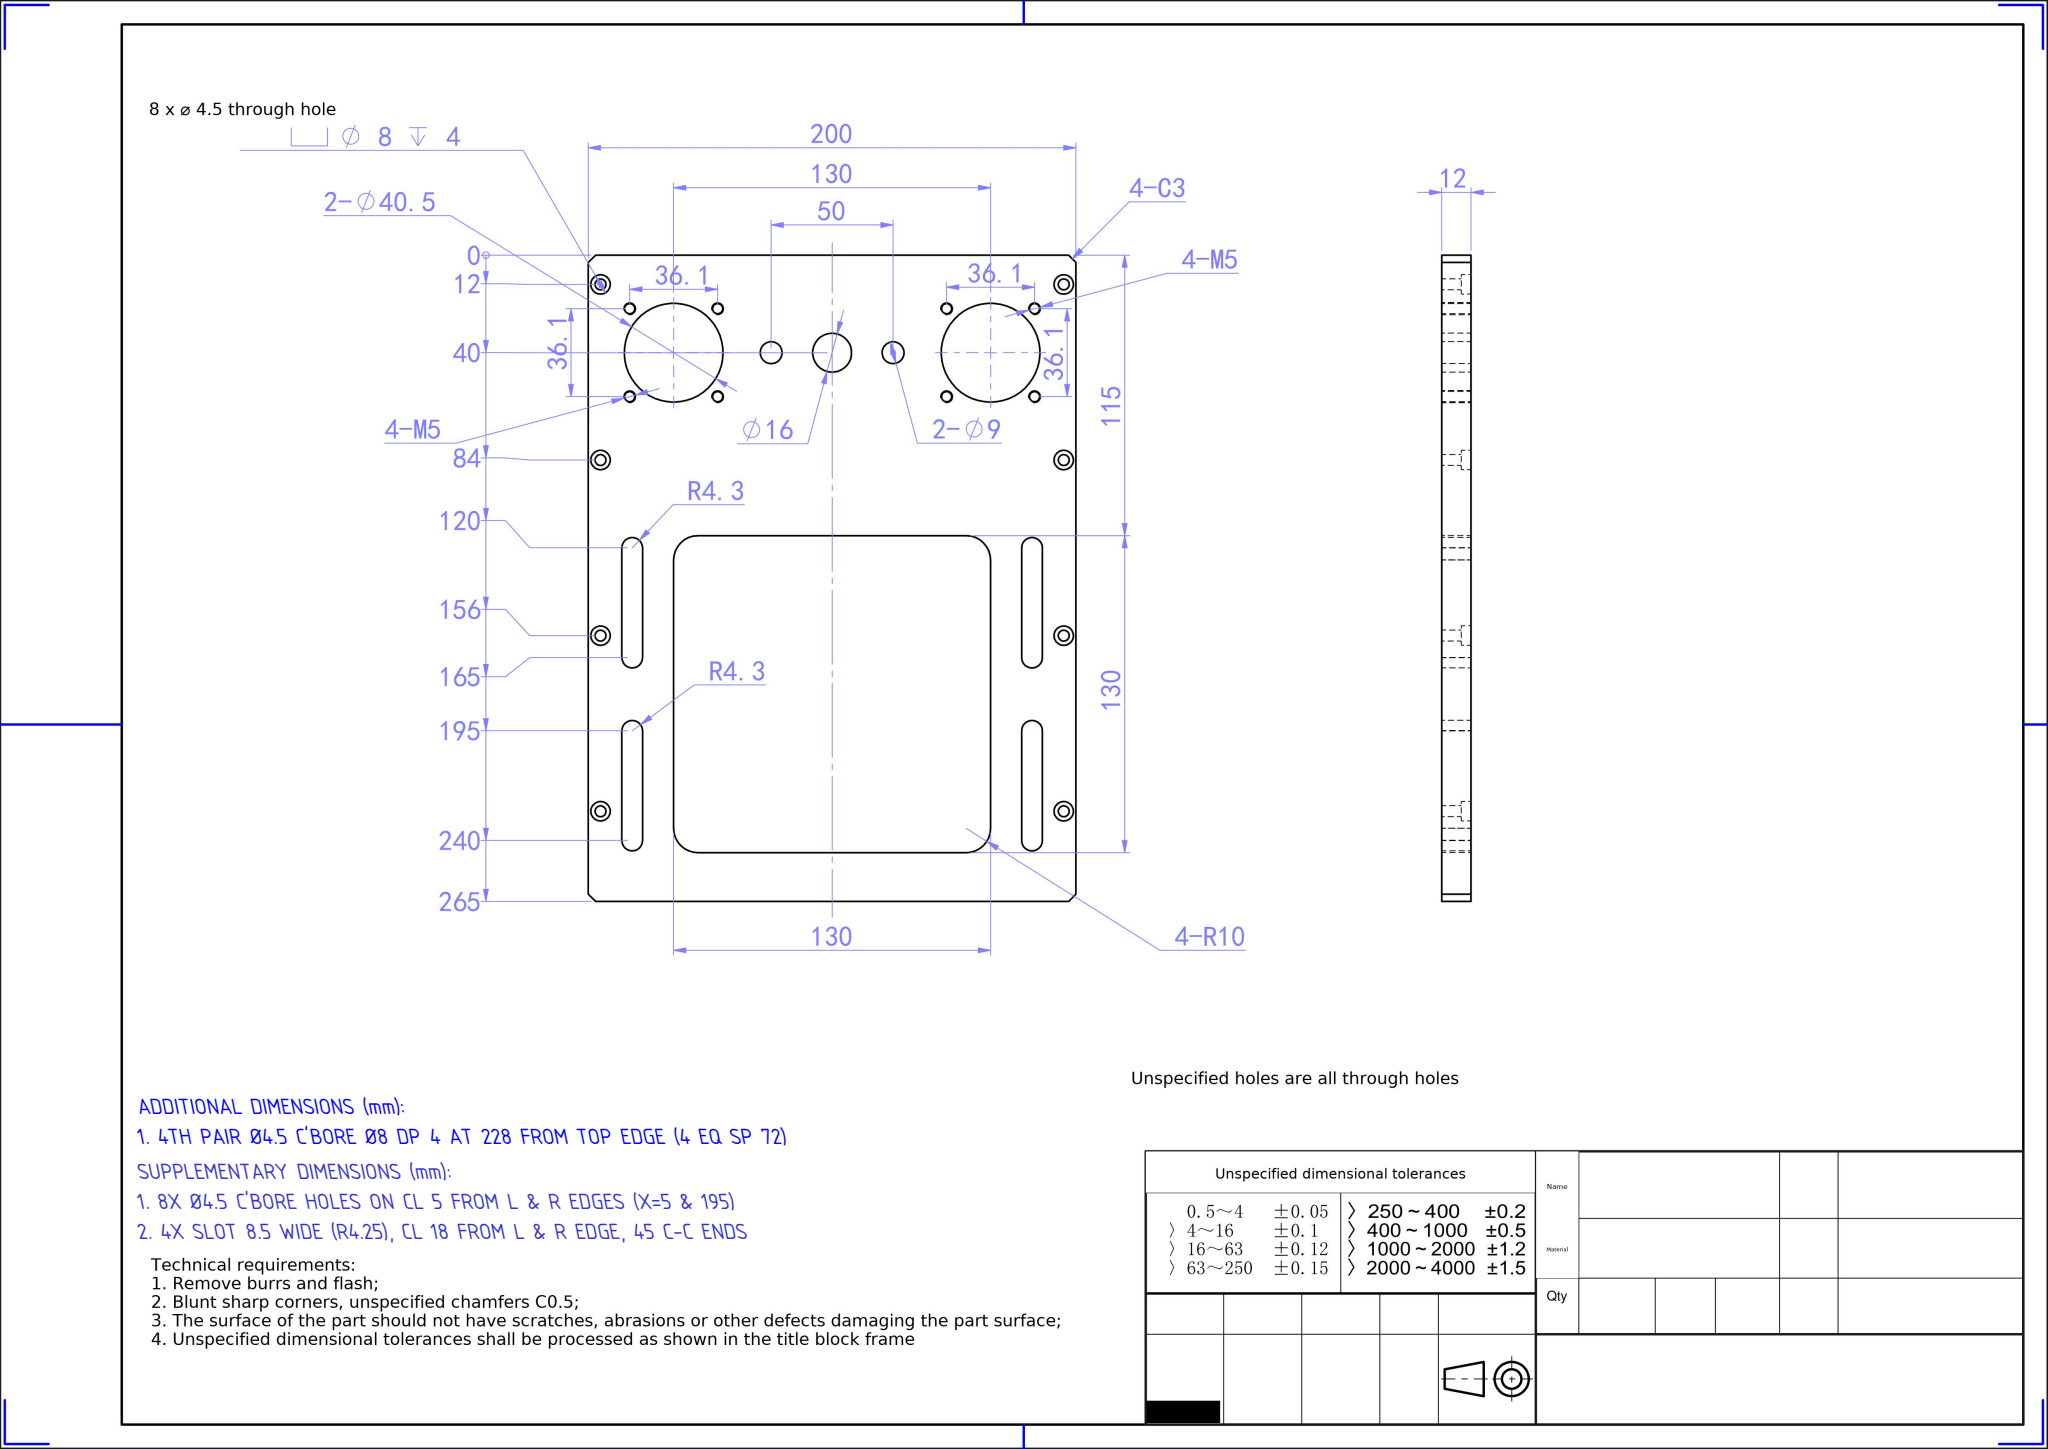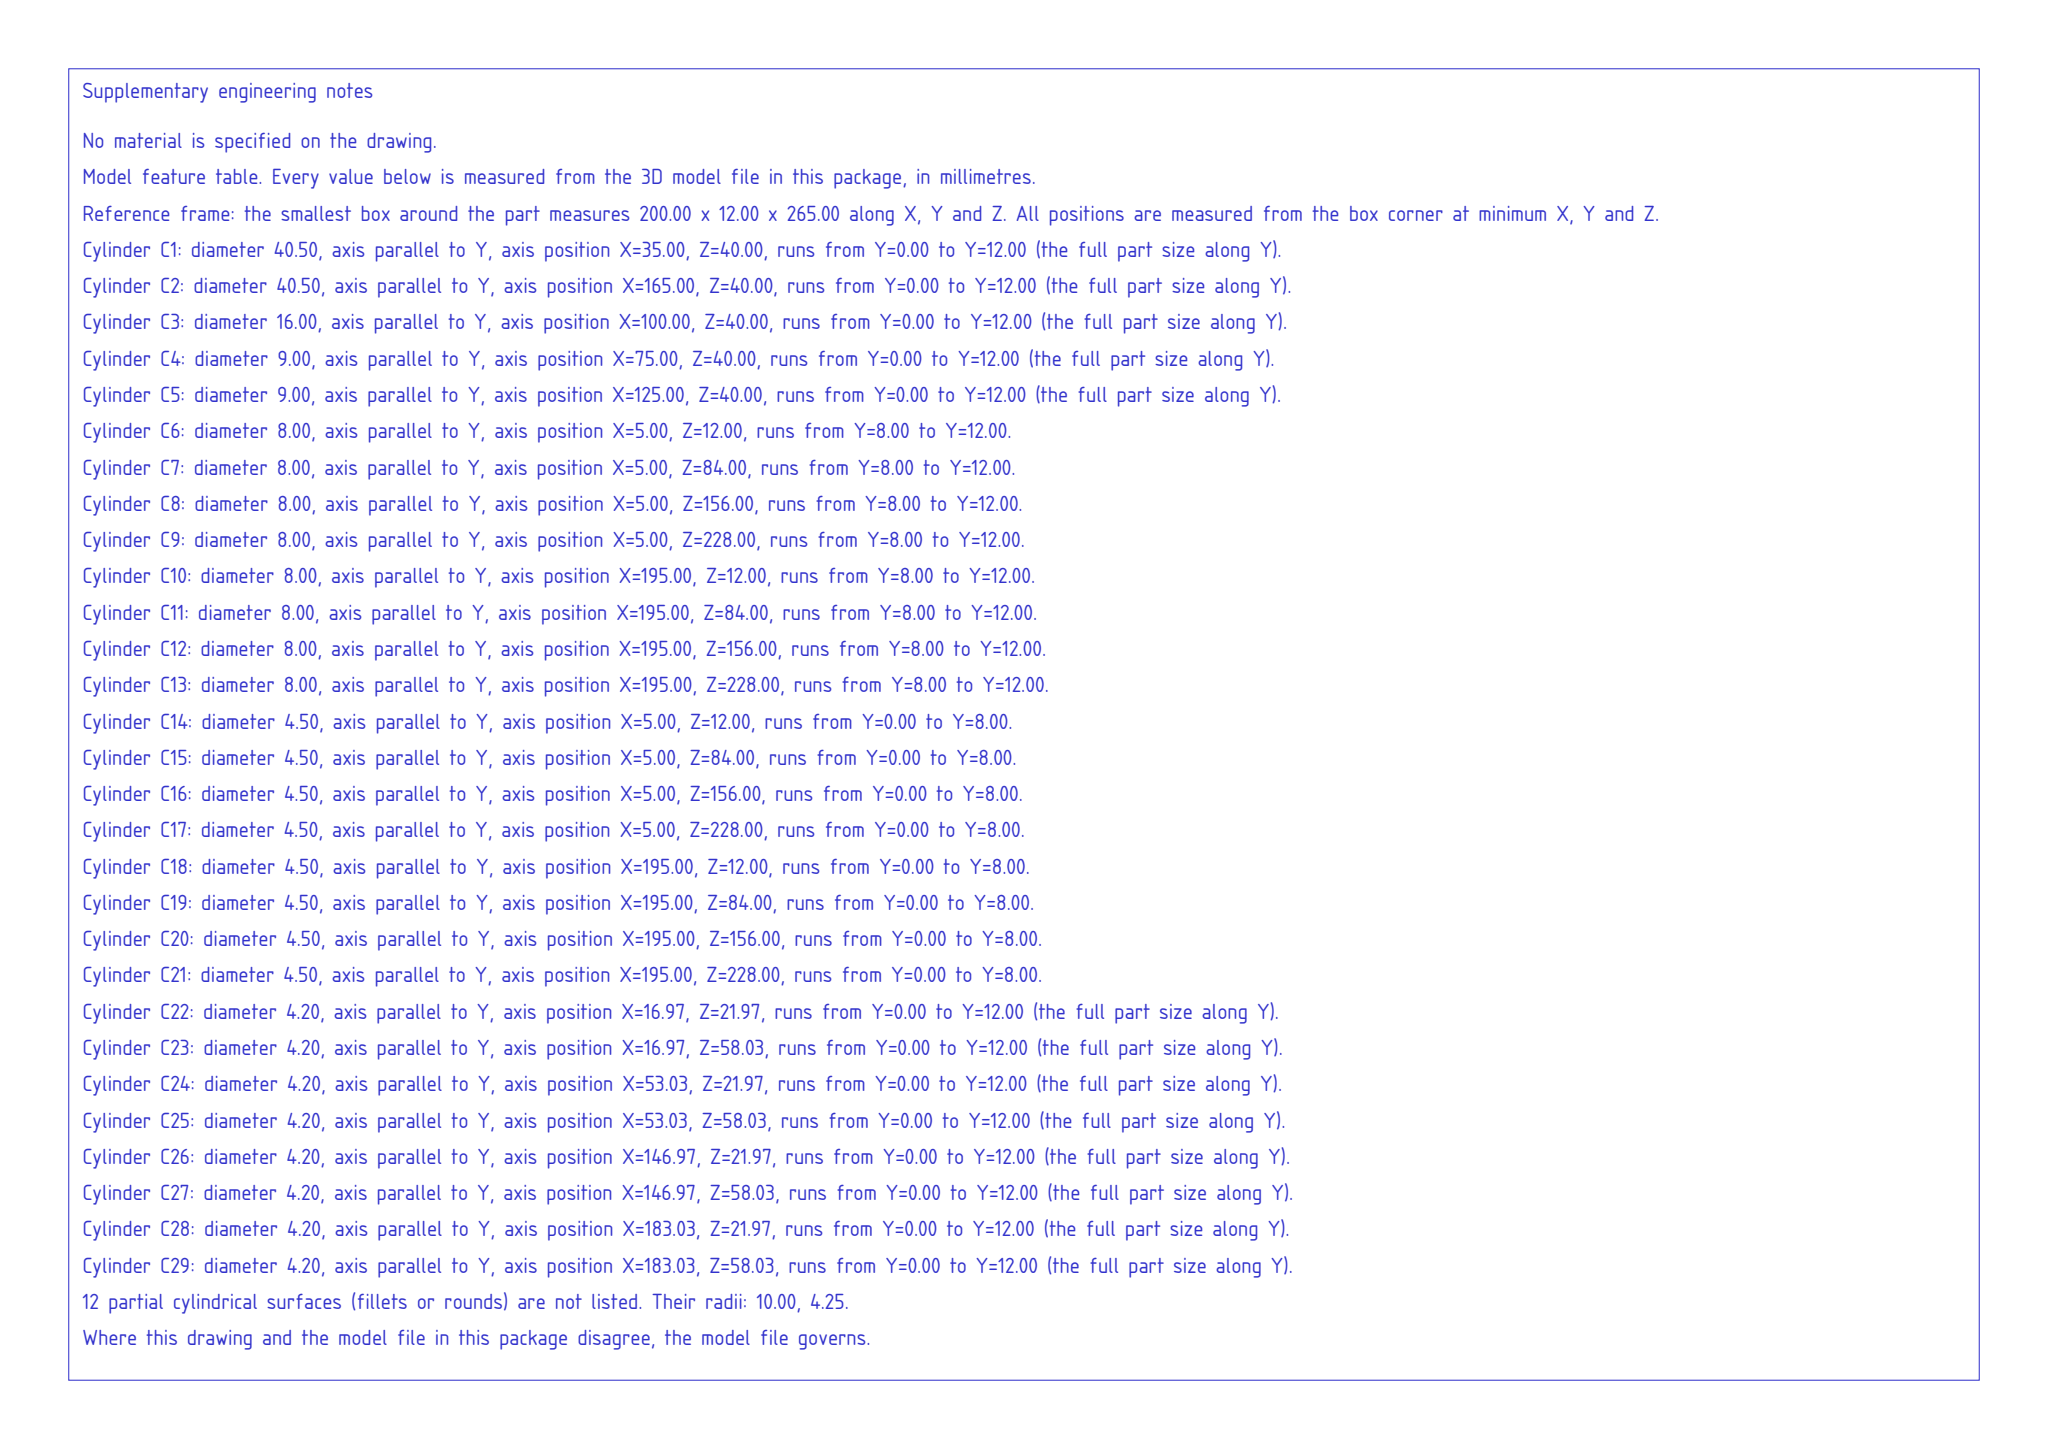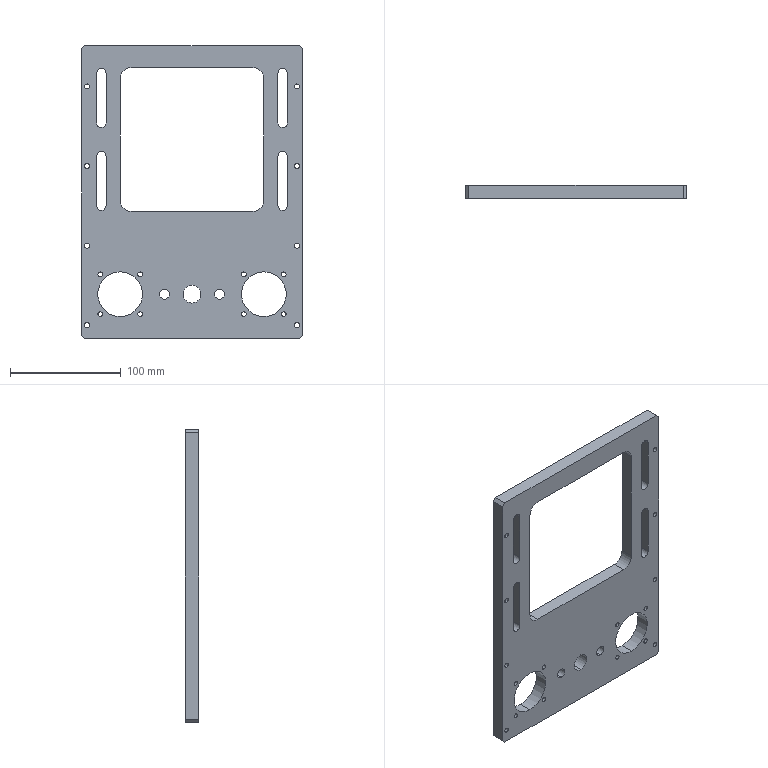Part | SolidWorks | mm | 1 solid | 104 faces | box 200 x 12 x 265 mm | volume 374116 mm3 | cylinder 74 | plane 30 | commonest cylinder face diameters 8 x16 4.5 x16 4.2 x16 8.5 x12 9 x4 40.5 x4 20 x4 16 x2
build123d program:
from build123d import *

# Parameters (mm, degrees)
SKETCH1_W                                       = 200
SKETCH1_H                                       = 265
SKETCH1_R                                       = 20.25
SKETCH1_R_2                                     = 8
SKETCH1_W_2                                     = 130
SKETCH1_H_2                                     = 130
EXTRUDE1_DEPTH                                  = 12
FILLET1_R                                       = 10
EXTRUDE2_DEPTH                                  = 324.735
SKETCH3_R                                       = 4.5
EXTRUDE3_DEPTH                                  = 324.735
SKETCH5_R                                       = 1
EXTRUDE4_DEPTH                                  = 324.735
M5_TAPPED_HOLE1_D                               = 4.2
M4_HEX_SOCKET_HEAD_CAP_SCREW_CBORE1_D           = 4.5
M4_HEX_SOCKET_HEAD_CAP_SCREW_CBORE1_CBORE_D     = 8
M4_HEX_SOCKET_HEAD_CAP_SCREW_CBORE1_CBORE_DEPTH = 4
CHAMFER1_SIZE                                   = 3


with BuildPart() as part:
    # Sketch1 → Extrude1 (new body)
    with BuildSketch(Plane(origin=(0, 0, 0), x_dir=(1, 0, 0), z_dir=(0, 1, 0))):
        with Locations((65.05, 145.742)):
            Rectangle(SKETCH1_W, SKETCH1_H)
        with Locations(Location((0.05031, 238.242, 0), (0, 0, 270))):
            Circle(SKETCH1_R, mode=Mode.SUBTRACT)
        with Locations(Location((130.05, 238.242, 0), (0, 0, 270))):
            Circle(SKETCH1_R, mode=Mode.SUBTRACT)
        with Locations(Location((65.05, 238.242, 0), (0, 0, 270))):
            Circle(SKETCH1_R_2, mode=Mode.SUBTRACT)
        with Locations((65.05, 98.242)):
            Rectangle(SKETCH1_W_2, SKETCH1_H_2, mode=Mode.SUBTRACT)
    extrude(amount=EXTRUDE1_DEPTH)

    # Fillet1
    fillet1_edges = [part.edges().sort_by_distance(p)[0] for p in [
        (0.05031, 6, -163.242),
        (0.05031, 6, -33.242),
        (130.05, 6, -33.242),
        (130.05, 6, -163.242),
    ]]
    fillet(fillet1_edges, radius=FILLET1_R)

    # Sketch2 → Extrude2 (cut, through all)
    with BuildSketch(Plane(origin=(0, 12, 0), x_dir=(-1, 0, 0), z_dir=(0, 1, 0))):
        with BuildLine():
            Line((-151.3, -83.242), (-151.3, -38.242))
            ThreePointArc((-151.3, -38.242), (-147.05, -33.992), (-142.8, -38.242))
            Line((-142.8, -38.242), (-142.8, -83.242))
            ThreePointArc((-142.8, -83.242), (-147.05, -87.492), (-151.3, -83.242))
        make_face()
        with BuildLine():
            Line((21.2, -158.242), (21.2, -113.242))
            ThreePointArc((21.2, -113.242), (16.95, -108.992), (12.7, -113.242))
            Line((12.7, -113.242), (12.7, -158.242))
            ThreePointArc((12.7, -158.242), (16.95, -162.492), (21.2, -158.242))
        make_face()
        with BuildLine():
            Line((12.7, -83.242), (12.7, -38.242))
            ThreePointArc((12.7, -38.242), (16.95, -33.992), (21.2, -38.242))
            Line((21.2, -38.242), (21.2, -83.242))
            ThreePointArc((21.2, -83.242), (16.95, -87.492), (12.7, -83.242))
        make_face()
        with BuildLine():
            Line((-142.8, -158.242), (-142.8, -113.242))
            ThreePointArc((-142.8, -113.242), (-147.05, -108.992), (-151.3, -113.242))
            Line((-151.3, -113.242), (-151.3, -158.242))
            ThreePointArc((-151.3, -158.242), (-147.05, -162.492), (-142.8, -158.242))
        make_face()
    extrude(amount=-EXTRUDE2_DEPTH, mode=Mode.SUBTRACT)

    # Sketch3 → Extrude3 (cut, through all)
    with BuildSketch(Plane(origin=(0, 12, 0), x_dir=(-1, 0, 0), z_dir=(0, 1, 0))):
        with Locations(Location((-40.05, -238.242, 0), (0, 0, 90))):
            Circle(SKETCH3_R)
        with Locations(Location((-90.05, -238.242, 0), (0, 0, 90))):
            Circle(SKETCH3_R)
    extrude(amount=-EXTRUDE3_DEPTH, mode=Mode.SUBTRACT)

    # Sketch5 → Extrude4 (cut, through all)
    with BuildSketch(Plane(origin=(0, 12, 0), x_dir=(-1, 0, 0), z_dir=(0, 1, 0))):
        with Locations(Location((-18.082, -220.211, 0), (0, 0, 90))):
            Circle(SKETCH5_R)
        with Locations(Location((-112.019, -220.211, 0), (0, 0, 90))):
            Circle(SKETCH5_R)
        with Locations(Location((17.981, -220.211, 0), (0, 0, 90))):
            Circle(SKETCH5_R)
        with Locations(Location((17.981, -256.273, 0), (0, 0, 90))):
            Circle(SKETCH5_R)
        with Locations(Location((-18.082, -256.273, 0), (0, 0, 90))):
            Circle(SKETCH5_R)
        with Locations(Location((-112.019, -256.273, 0), (0, 0, 90))):
            Circle(SKETCH5_R)
        with Locations(Location((-148.082, -256.273, 0), (0, 0, 90))):
            Circle(SKETCH5_R)
        with Locations(Location((-148.082, -220.211, 0), (0, 0, 90))):
            Circle(SKETCH5_R)
    extrude(amount=-EXTRUDE4_DEPTH, mode=Mode.SUBTRACT)

    # M5 Tapped Hole1 (through all)
    with Locations(Plane(origin=(-17.981, 12, -256.273), x_dir=(0, 0, 1), z_dir=(0, 1, 0))):
        with Locations((0, 0), (0, 36.062), (36.062, 0), (36.062, 36.062), (0, 166.062), (0, 130), (36.062, 130), (36.062, 166.062)):
            Hole(M5_TAPPED_HOLE1_D / 2)

    # M4 Hex Socket Head Cap Screw CBORE1 (through all)
    with Locations(Plane(origin=(160.05, 12, -266.242), x_dir=(0, 0, 1), z_dir=(0, 1, 0))):
        with Locations((0, 0), (72, 0), (144, 0), (216, 0), (216, -190), (144, -190), (72, -190), (0, -190)):
            CounterBoreHole(M4_HEX_SOCKET_HEAD_CAP_SCREW_CBORE1_D / 2, M4_HEX_SOCKET_HEAD_CAP_SCREW_CBORE1_CBORE_D / 2, M4_HEX_SOCKET_HEAD_CAP_SCREW_CBORE1_CBORE_DEPTH)

    # Chamfer1
    chamfer1_edges = [part.edges().sort_by_distance(p)[0] for p in [
        (-34.95, 6, -278.242),
        (165.05, 6, -278.242),
        (165.05, 6, -13.242),
        (-34.95, 6, -13.242),
    ]]
    chamfer(chamfer1_edges, length=CHAMFER1_SIZE)


solid = part.part